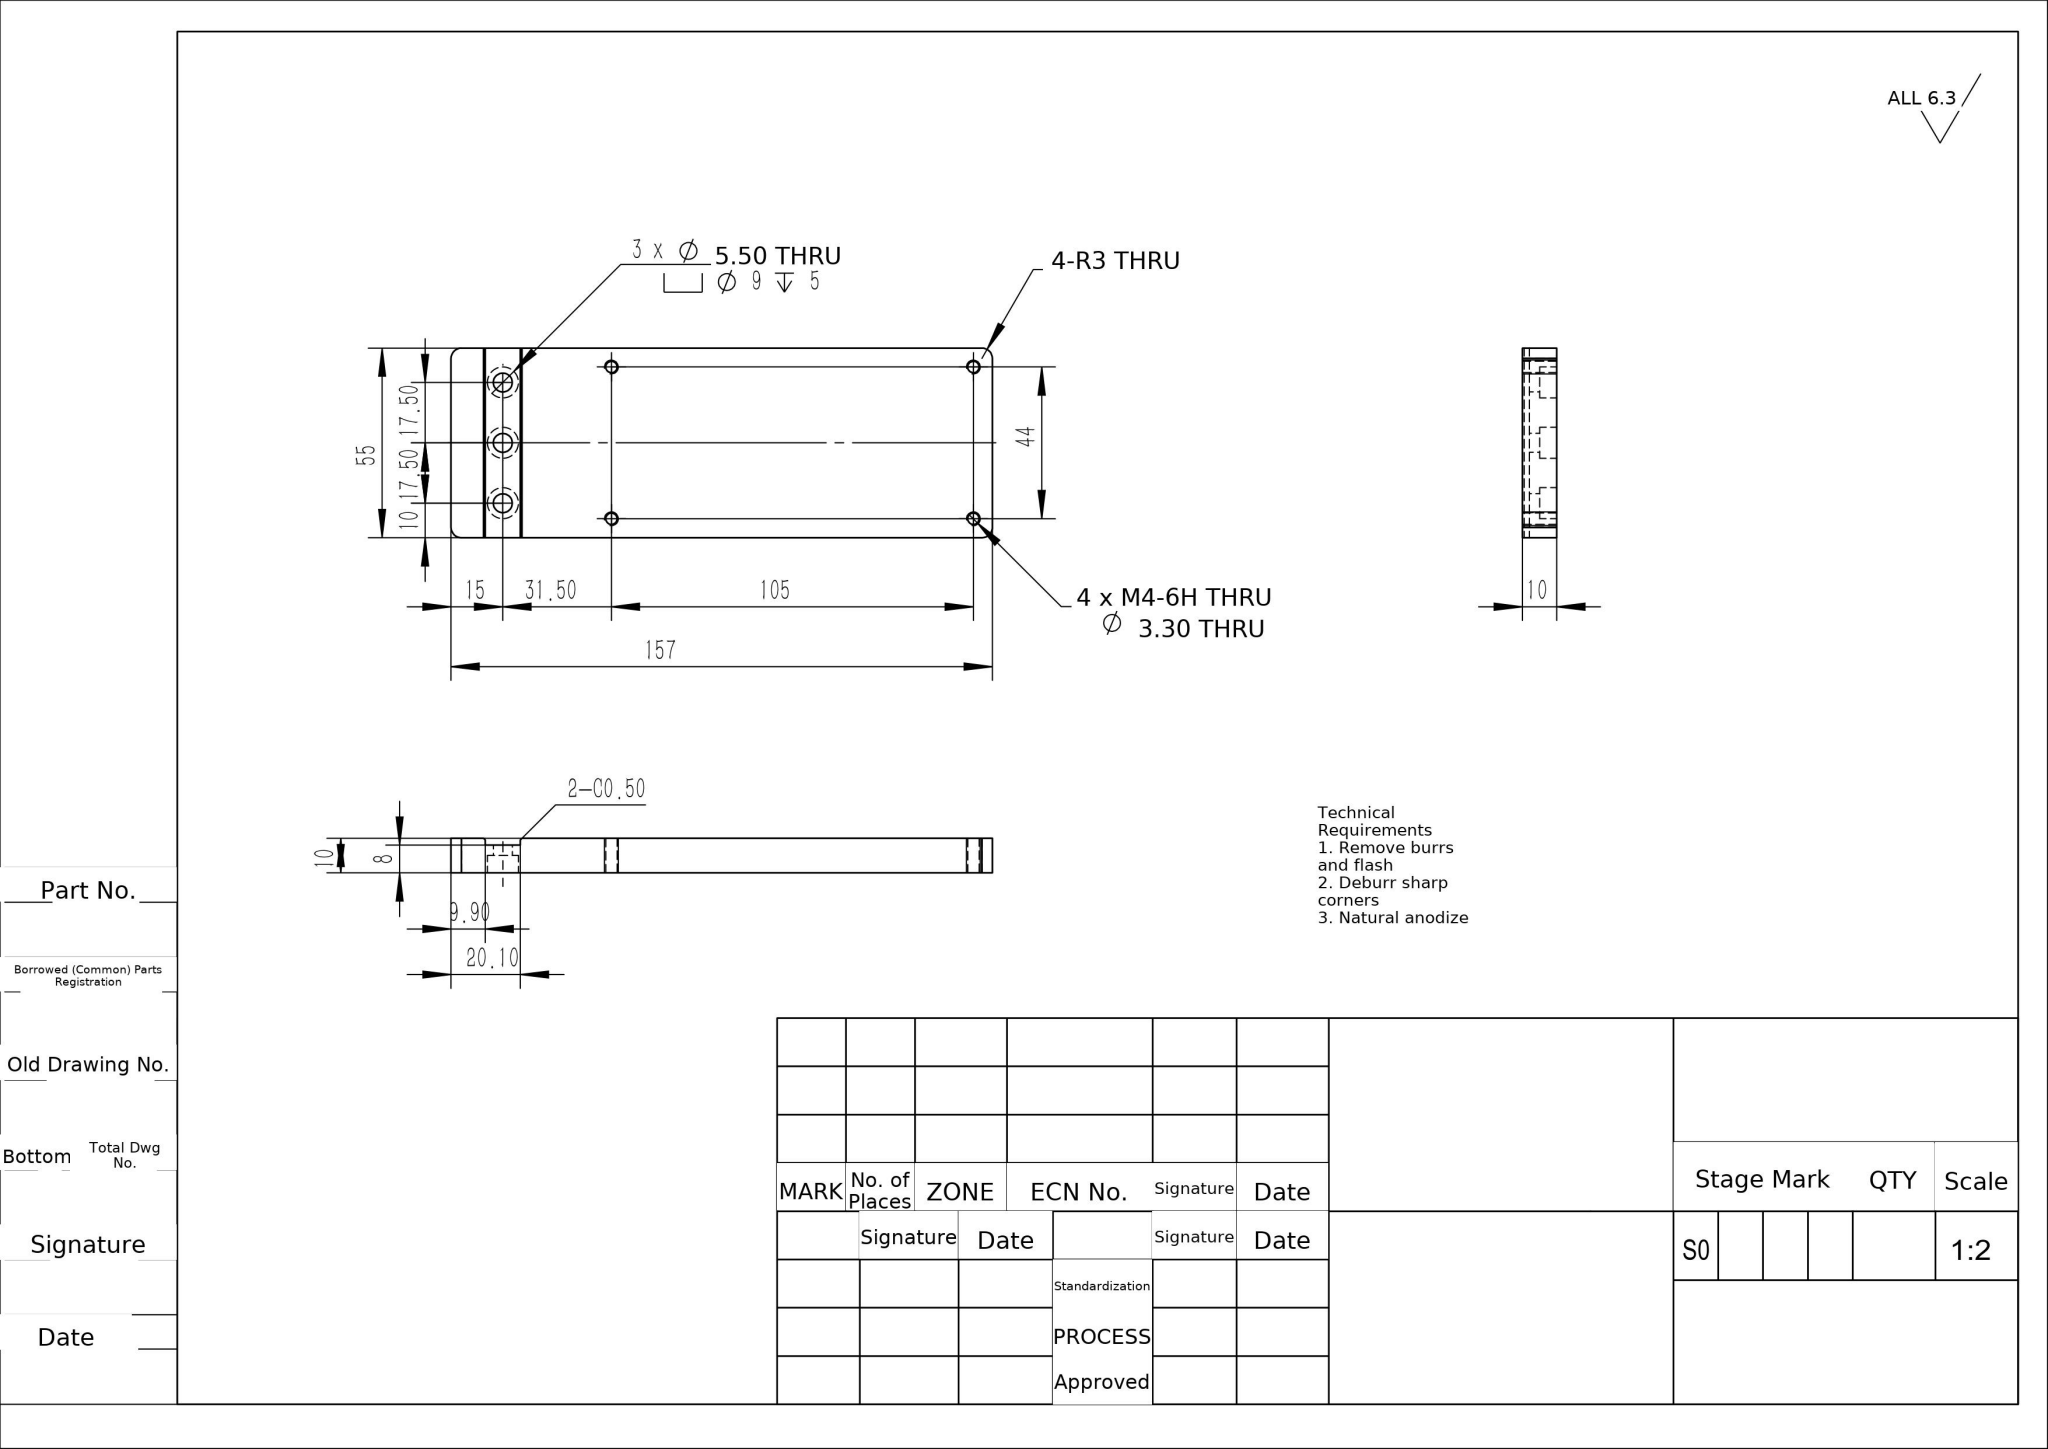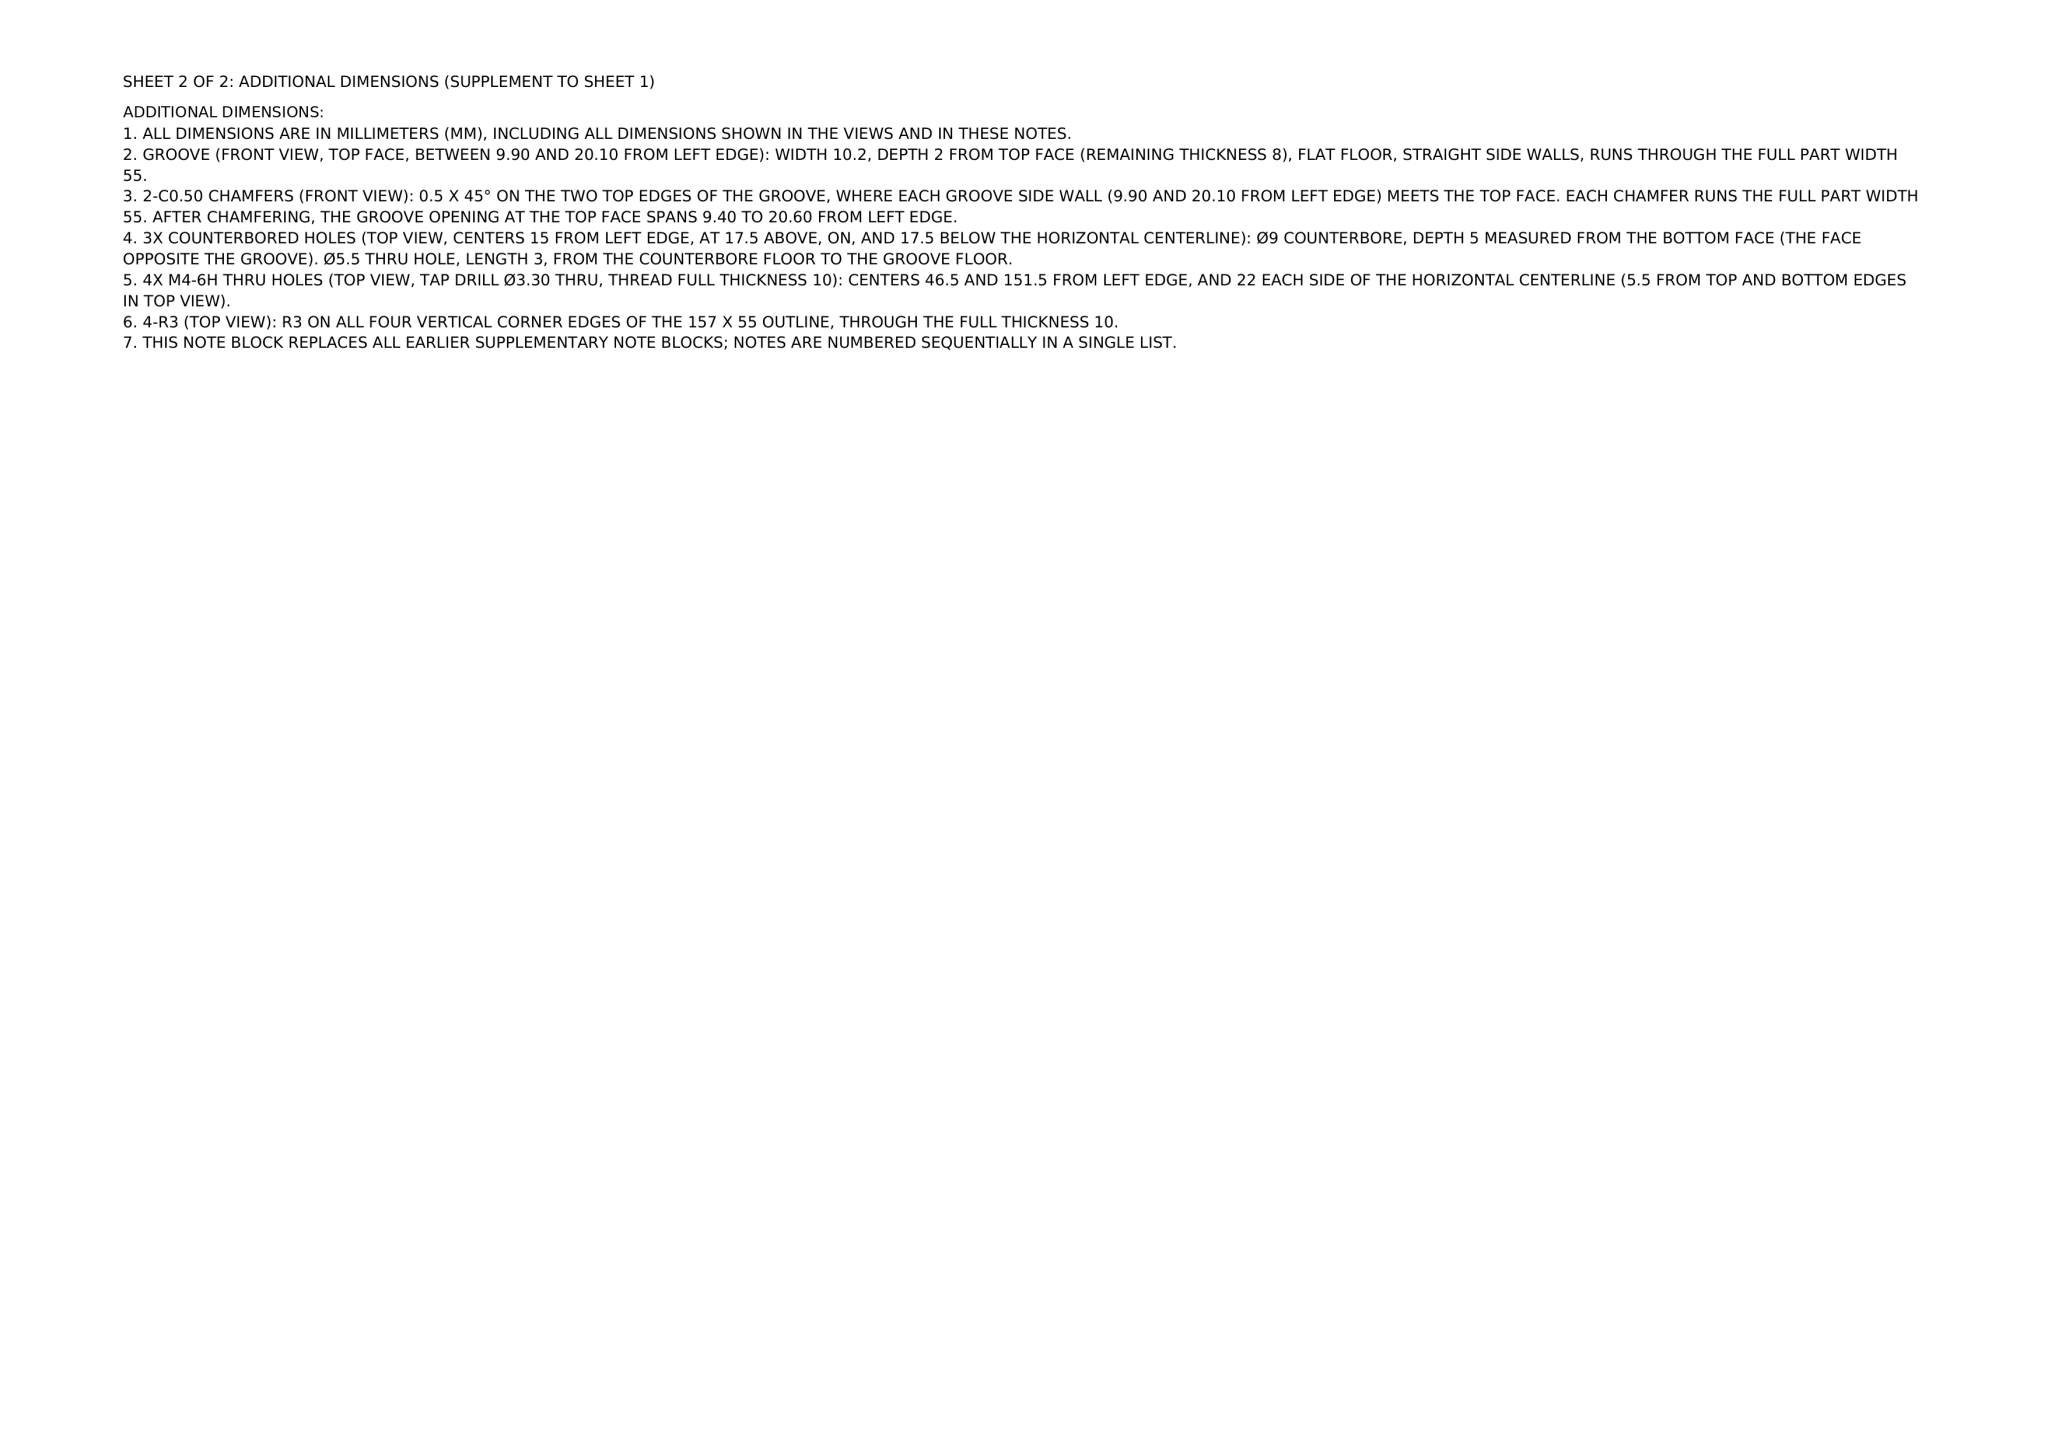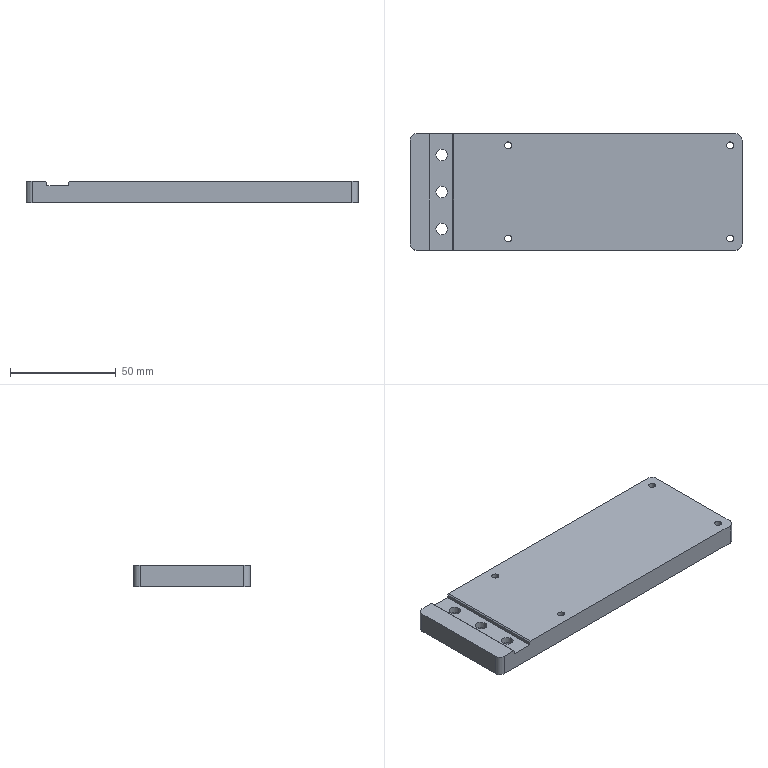Part | NX | mm | 1 solid | 39 faces | box 157 x 55 x 10 mm | volume 83627 mm3 | cylinder 24 | plane 15 | commonest cylinder face diameters 3.3 x8 9 x6 5.5 x6 6 x4